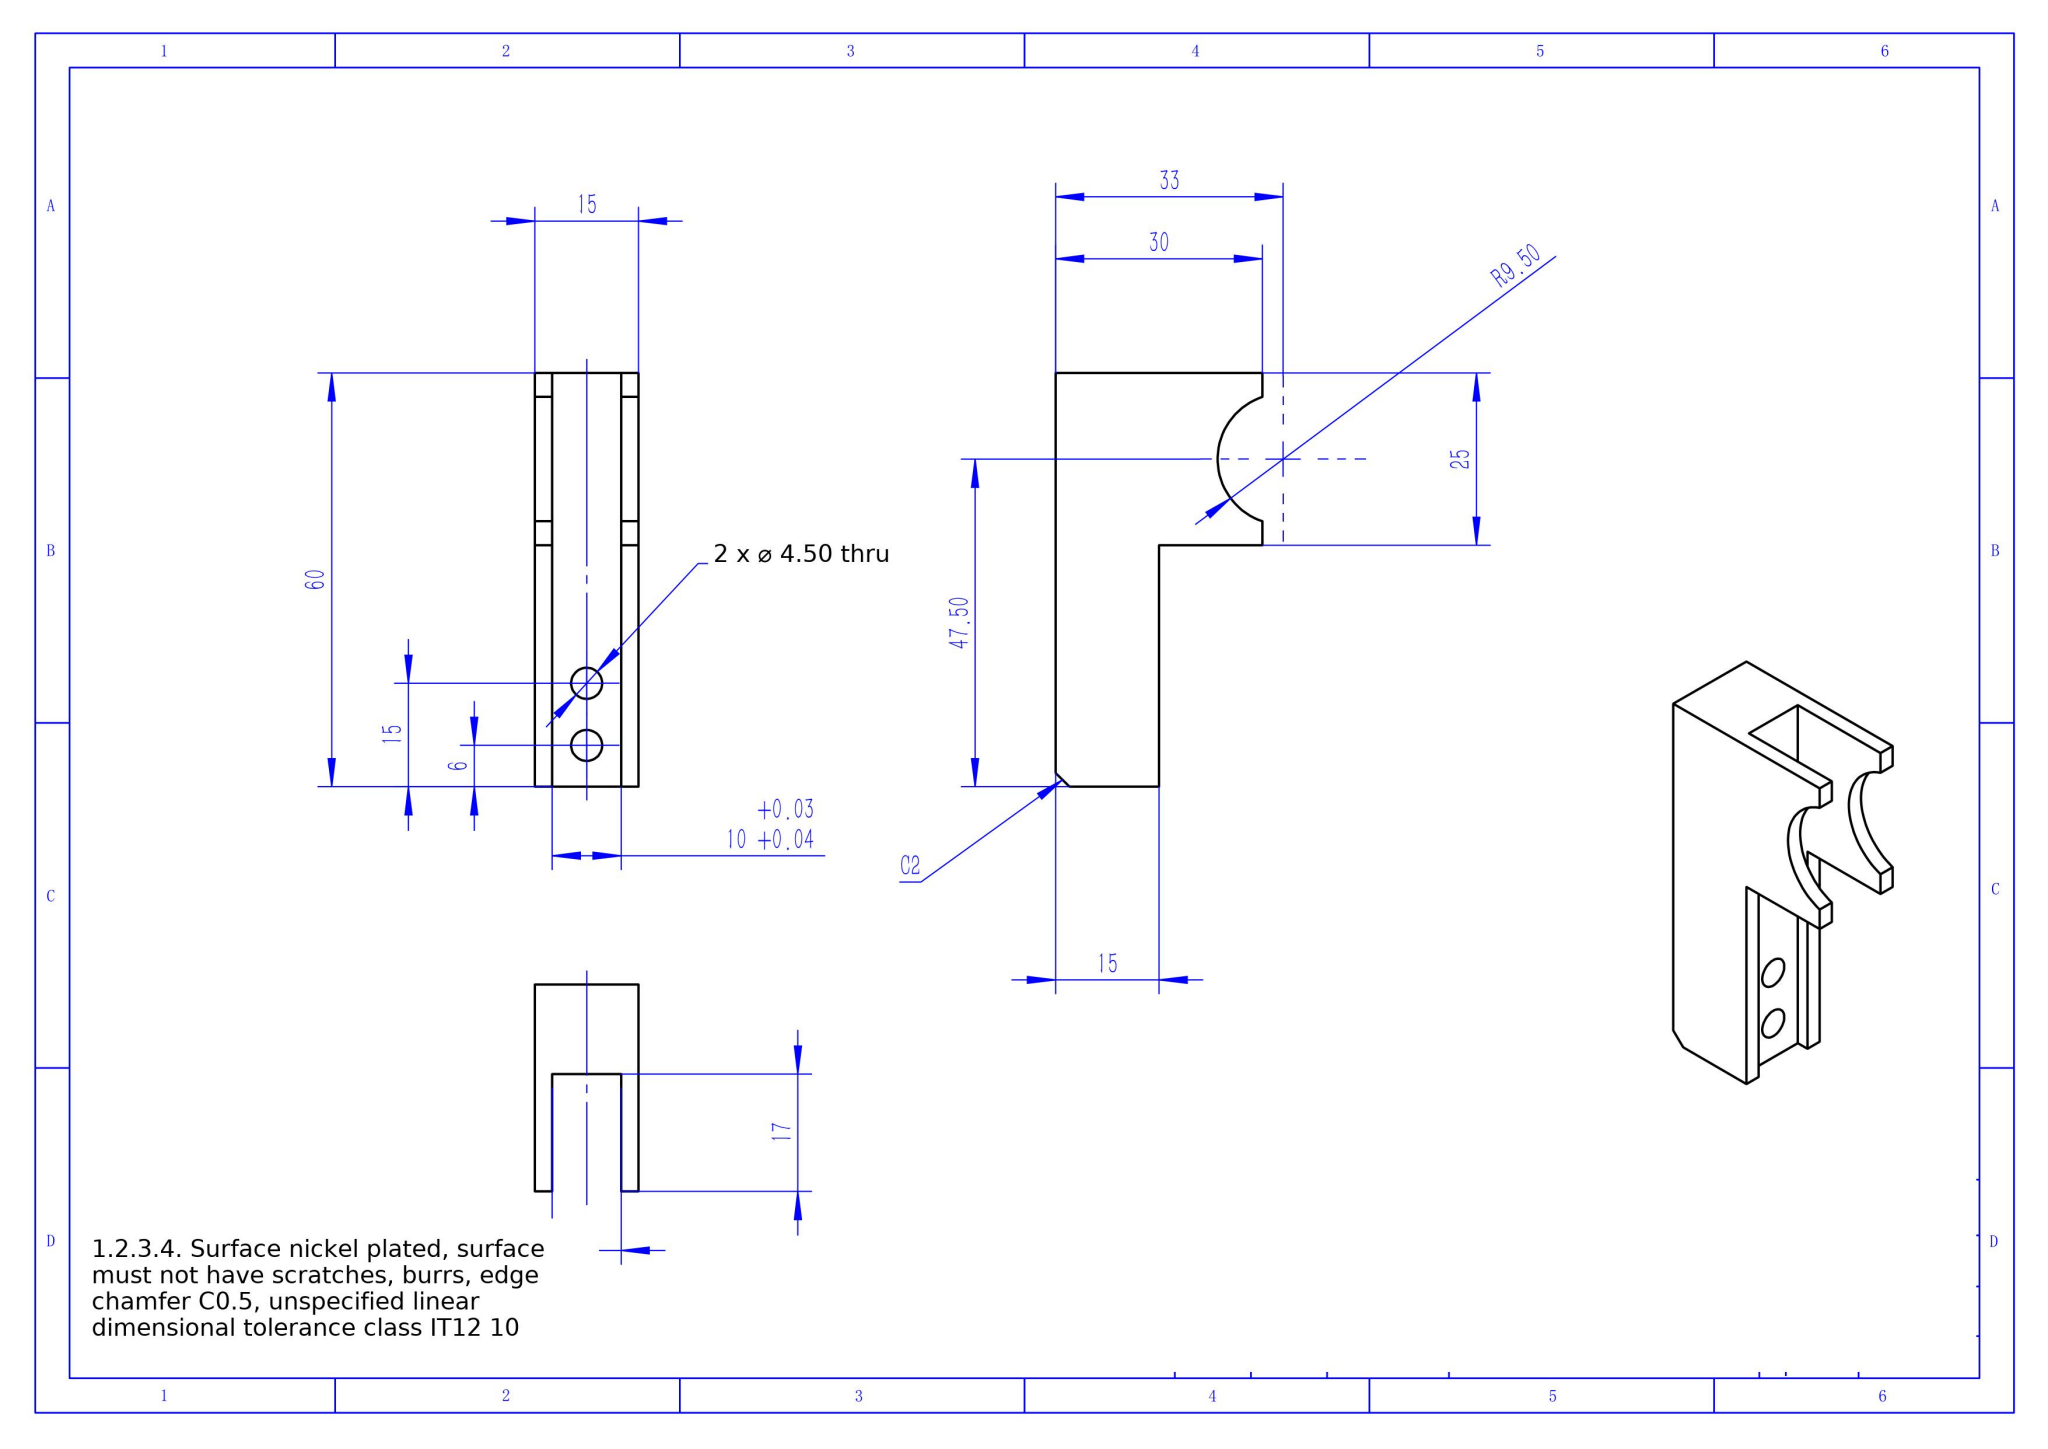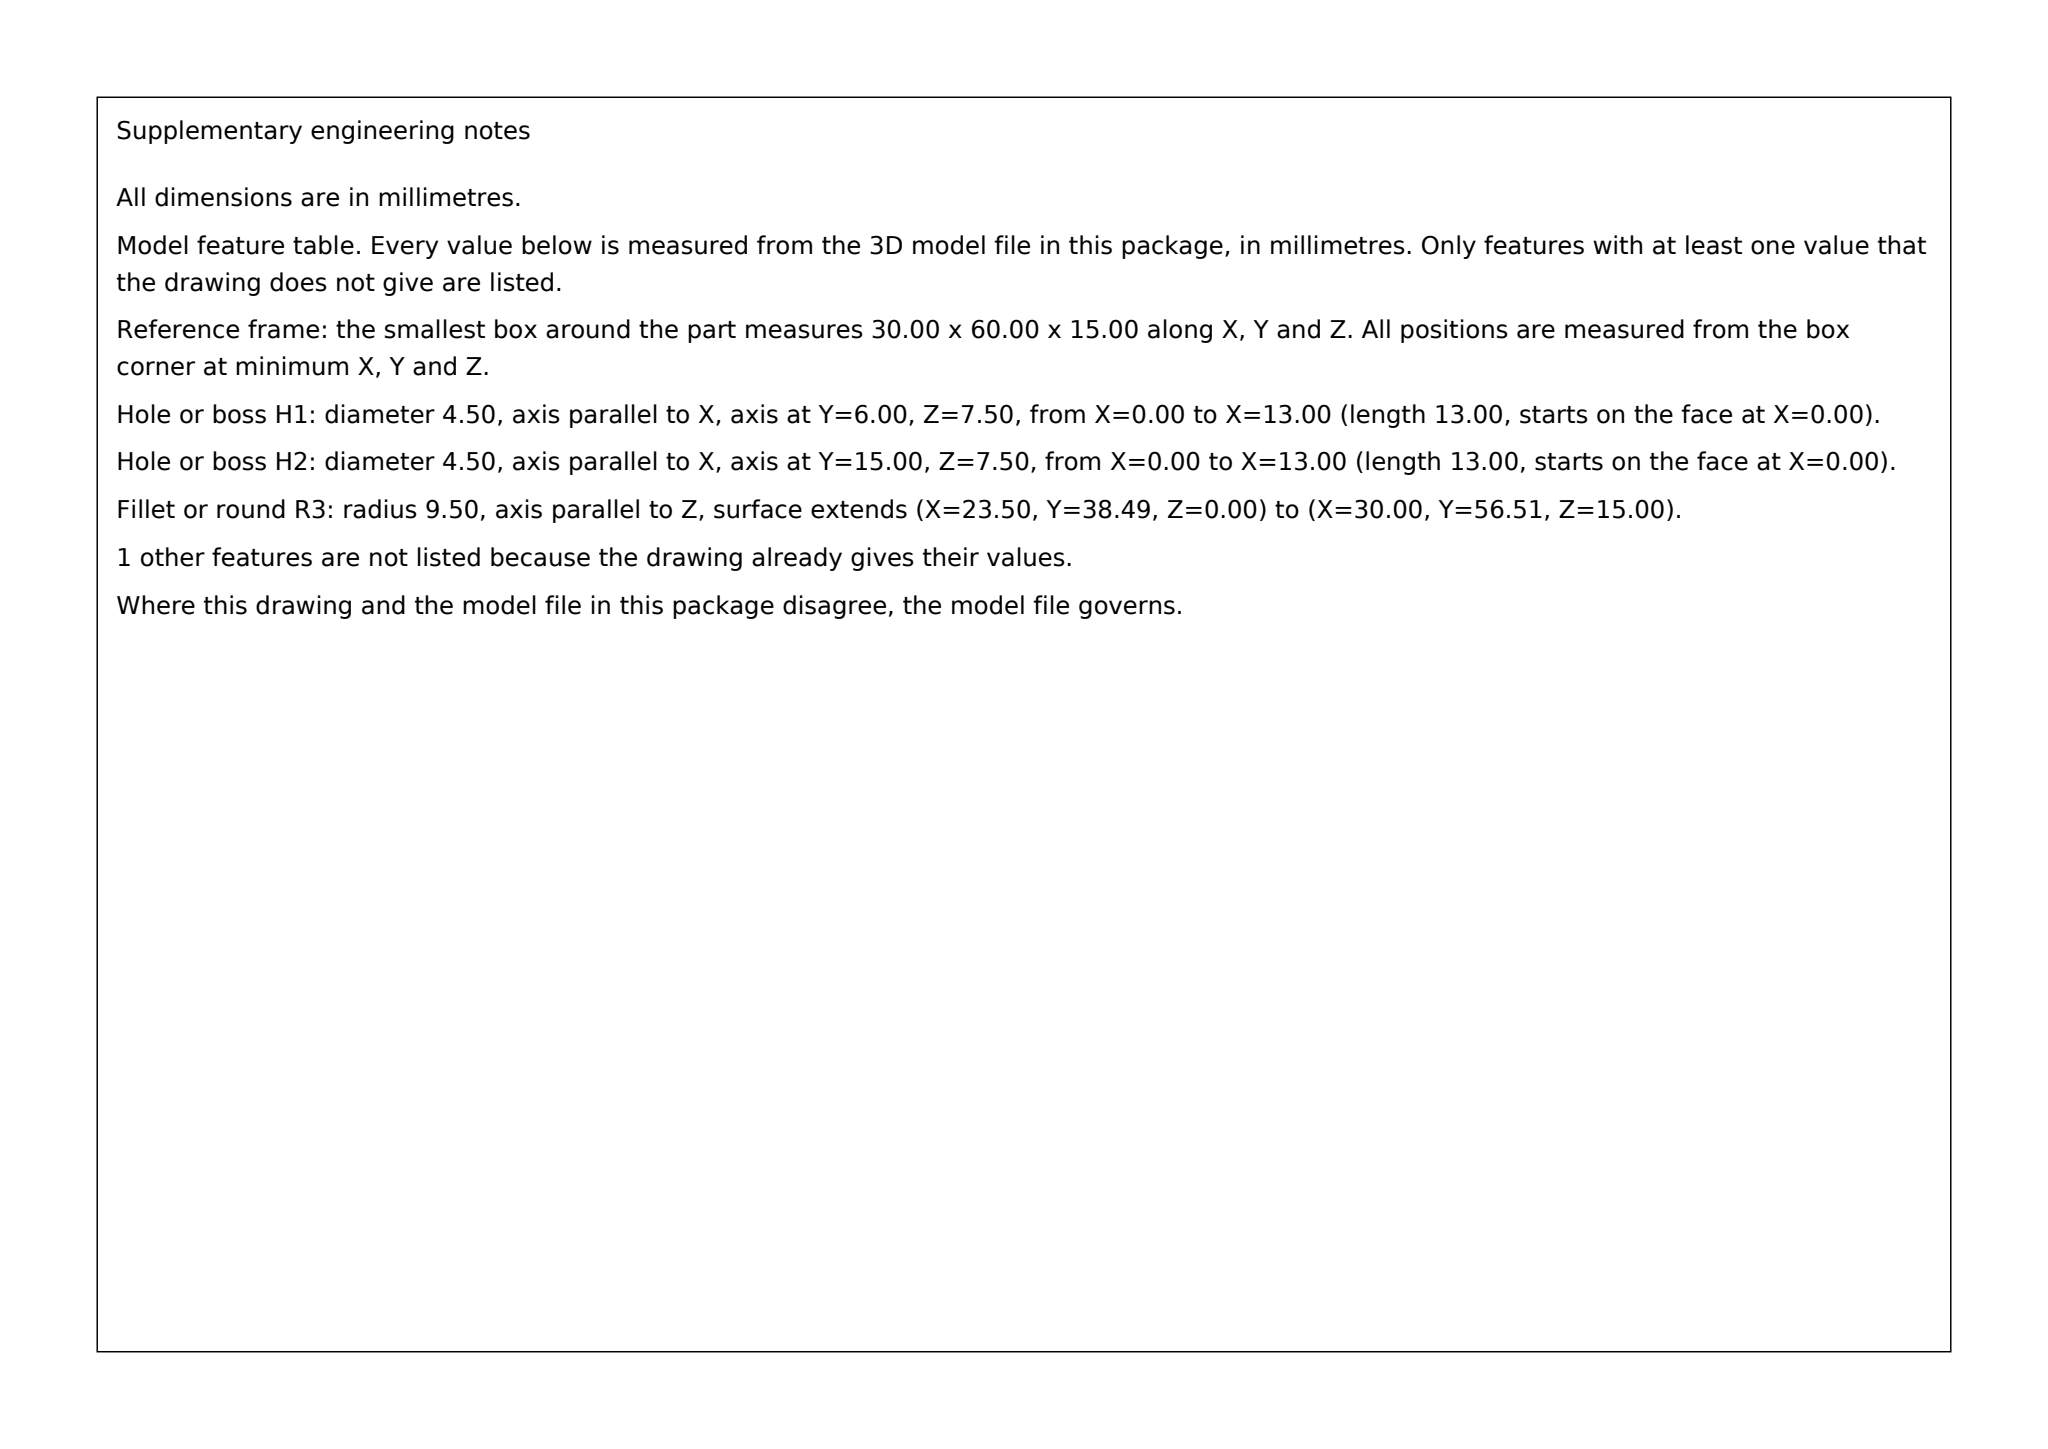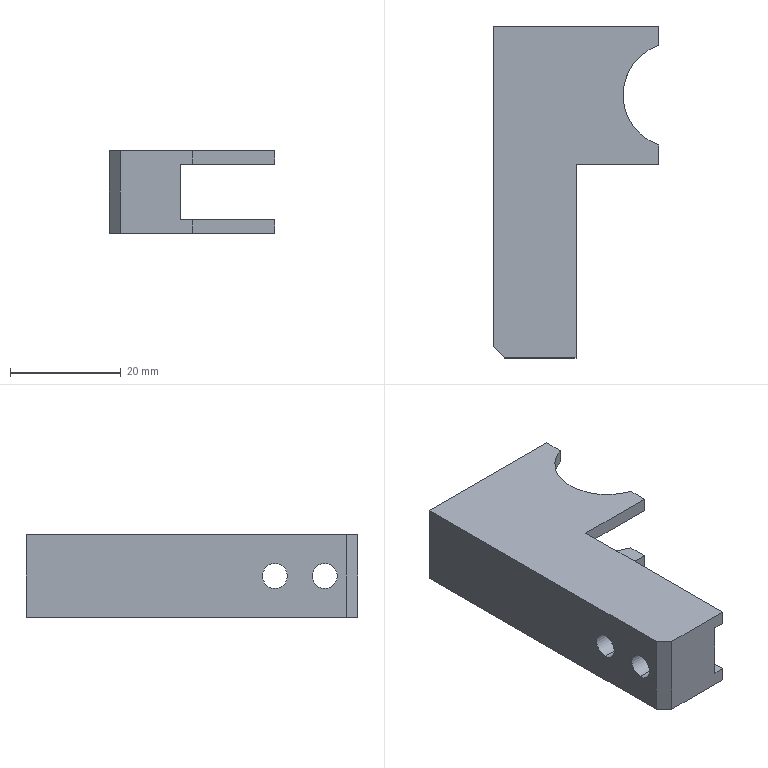Part | SolidWorks | mm | 1 solid | 25 faces | box 30 x 60 x 15 mm | volume 13303 mm3 | plane 17 | cylinder 8 | commonest cylinder face diameters 19 x4 4.5 x4
build123d program:
from build123d import *

# Parameters (mm, degrees)
BOSS_EXTRUDE1_DEPTH        = 15
F_4_5_4_5_DIAMETER_HOLE1_D = 4.5
CHAMFER1_SIZE              = 2
SKETCH5_W                  = 10
SKETCH5_H                  = 124.839
CUT_EXTRUDE2_DEPTH         = 17


with BuildPart() as part:
    # Sketch1 → Boss-Extrude1 (new body)
    with BuildSketch(Plane.XY):
        with BuildLine():
            Line((0, 0), (15, 0))
            Line((15, 0), (15, 35))
            Line((15, 35), (30, 35))
            Line((30, 35), (30, 38.486))
            ThreePointArc((30, 38.486), (23.5, 47.5), (30, 56.514))
            Line((30, 56.514), (30, 60))
            Line((30, 60), (0, 60))
            Line((0, 60), (0, 0))
        make_face()
    extrude(amount=BOSS_EXTRUDE1_DEPTH)

    # 4.5 _4.5_ Diameter Hole1 (through all)
    with Locations(Plane.ZY):
        with Locations((7.5, 6), (7.5, 15)):
            Hole(F_4_5_4_5_DIAMETER_HOLE1_D / 2)

    # Chamfer1
    chamfer1_edges = [part.edges().sort_by_distance(p)[0] for p in [
        (0, 0, 7.5),
    ]]
    chamfer(chamfer1_edges, length=CHAMFER1_SIZE)

    # Sketch5 → Cut-Extrude2 (cut)
    with BuildSketch(Plane(origin=(30, 0, 0), x_dir=(0, 0, -1), z_dir=(1, 0, 0))):
        with Locations((-7.5, 60)):
            Rectangle(SKETCH5_W, SKETCH5_H)
    extrude(amount=-CUT_EXTRUDE2_DEPTH, mode=Mode.SUBTRACT)


solid = part.part
STEP:
#1=CARTESIAN_POINT('',(23.5,47.5,15.));
#2=VERTEX_POINT('',#1);
#3=CARTESIAN_POINT('',(30.,56.514,15.));
#4=VERTEX_POINT('',#3);
#5=CARTESIAN_POINT('',(33.,47.5,15.));
#6=DIRECTION('',(0.,0.,-1.));
#7=DIRECTION('',(1.,0.,0.));
#8=AXIS2_PLACEMENT_3D('',#5,#6,#7);
#9=CIRCLE('',#8,9.5);
#10=EDGE_CURVE('',#2,#4,#9,.T.);
#11=ORIENTED_EDGE('',*,*,#10,.F.);
#12=CARTESIAN_POINT('',(23.5,47.5,12.5));
#13=VERTEX_POINT('',#12);
#14=CARTESIAN_POINT('',(23.5,47.5,15.));
#15=DIRECTION('',(0.,0.,-1.));
#16=VECTOR('',#15,1000.);
#17=LINE('',#14,#16);
#18=EDGE_CURVE('',#2,#13,#17,.T.);
#19=ORIENTED_EDGE('',*,*,#18,.T.);
#20=CARTESIAN_POINT('',(30.,56.514,12.5));
#21=VERTEX_POINT('',#20);
#22=CARTESIAN_POINT('',(33.,47.5,12.5));
#23=DIRECTION('',(0.,0.,-1.));
#24=DIRECTION('',(1.,-0.,0.));
#25=AXIS2_PLACEMENT_3D('',#22,#23,#24);
#26=CIRCLE('',#25,9.5);
#27=EDGE_CURVE('',#13,#21,#26,.T.);
#28=ORIENTED_EDGE('',*,*,#27,.T.);
#29=CARTESIAN_POINT('',(30.,56.514,15.));
#30=DIRECTION('',(0.,0.,-1.));
#31=VECTOR('',#30,1000.);
#32=LINE('',#29,#31);
#33=EDGE_CURVE('',#4,#21,#32,.T.);
#34=ORIENTED_EDGE('',*,*,#33,.F.);
#35=EDGE_LOOP('',(#11,#19,#28,#34));
#36=FACE_OUTER_BOUND('',#35,.T.);
#37=CARTESIAN_POINT('',(33.,47.5,15.));
#38=DIRECTION('',(0.,0.,-1.));
#39=DIRECTION('',(-1.,0.,0.));
#40=AXIS2_PLACEMENT_3D('',#37,#38,#39);
#41=CYLINDRICAL_SURFACE('',#40,9.5);
#42=ADVANCED_FACE('',(#36),#41,.F.);
#43=CARTESIAN_POINT('',(13.,6.,5.25));
#44=VERTEX_POINT('',#43);
#45=CARTESIAN_POINT('',(13.,6.,9.75));
#46=VERTEX_POINT('',#45);
#47=CARTESIAN_POINT('',(13.,6.,7.5));
#48=DIRECTION('',(-1.,0.,0.));
#49=DIRECTION('',(0.,0.,-1.));
#50=AXIS2_PLACEMENT_3D('',#47,#48,#49);
#51=CIRCLE('',#50,2.25);
#52=EDGE_CURVE('',#44,#46,#51,.T.);
#53=ORIENTED_EDGE('',*,*,#52,.F.);
#54=CARTESIAN_POINT('',(-0.,6.,5.25));
#55=VERTEX_POINT('',#54);
#56=CARTESIAN_POINT('',(0.,6.,5.25));
#57=DIRECTION('',(-1.,0.,0.));
#58=VECTOR('',#57,1000.);
#59=LINE('',#56,#58);
#60=EDGE_CURVE('',#44,#55,#59,.T.);
#61=ORIENTED_EDGE('',*,*,#60,.T.);
#62=CARTESIAN_POINT('',(-0.,6.,9.75));
#63=VERTEX_POINT('',#62);
#64=CARTESIAN_POINT('',(-0.,6.,7.5));
#65=DIRECTION('',(-1.,0.,0.));
#66=DIRECTION('',(0.,0.,1.));
#67=AXIS2_PLACEMENT_3D('',#64,#65,#66);
#68=CIRCLE('',#67,2.25);
#69=EDGE_CURVE('',#55,#63,#68,.T.);
#70=ORIENTED_EDGE('',*,*,#69,.T.);
#71=CARTESIAN_POINT('',(0.,6.,9.75));
#72=DIRECTION('',(-1.,0.,0.));
#73=VECTOR('',#72,1000.);
#74=LINE('',#71,#73);
#75=EDGE_CURVE('',#46,#63,#74,.T.);
#76=ORIENTED_EDGE('',*,*,#75,.F.);
#77=EDGE_LOOP('',(#53,#61,#70,#76));
#78=FACE_OUTER_BOUND('',#77,.T.);
#79=CARTESIAN_POINT('',(0.,6.,7.5));
#80=DIRECTION('',(-1.,0.,0.));
#81=DIRECTION('',(0.,0.,1.));
#82=AXIS2_PLACEMENT_3D('',#79,#80,#81);
#83=CYLINDRICAL_SURFACE('',#82,2.25);
#84=ADVANCED_FACE('',(#78),#83,.F.);
#85=CARTESIAN_POINT('',(13.,15.,5.25));
#86=VERTEX_POINT('',#85);
#87=CARTESIAN_POINT('',(13.,15.,9.75));
#88=VERTEX_POINT('',#87);
#89=CARTESIAN_POINT('',(13.,15.,7.5));
#90=DIRECTION('',(-1.,0.,0.));
#91=DIRECTION('',(0.,0.,-1.));
#92=AXIS2_PLACEMENT_3D('',#89,#90,#91);
#93=CIRCLE('',#92,2.25);
#94=EDGE_CURVE('',#86,#88,#93,.T.);
#95=ORIENTED_EDGE('',*,*,#94,.F.);
#96=CARTESIAN_POINT('',(-0.,15.,5.25));
#97=VERTEX_POINT('',#96);
#98=CARTESIAN_POINT('',(0.,15.,5.25));
#99=DIRECTION('',(-1.,0.,0.));
#100=VECTOR('',#99,1000.);
#101=LINE('',#98,#100);
#102=EDGE_CURVE('',#86,#97,#101,.T.);
#103=ORIENTED_EDGE('',*,*,#102,.T.);
#104=CARTESIAN_POINT('',(-0.,15.,9.75));
#105=VERTEX_POINT('',#104);
#106=CARTESIAN_POINT('',(-0.,15.,7.5));
#107=DIRECTION('',(-1.,0.,0.));
#108=DIRECTION('',(0.,0.,1.));
#109=AXIS2_PLACEMENT_3D('',#106,#107,#108);
#110=CIRCLE('',#109,2.25);
#111=EDGE_CURVE('',#97,#105,#110,.T.);
#112=ORIENTED_EDGE('',*,*,#111,.T.);
#113=CARTESIAN_POINT('',(0.,15.,9.75));
#114=DIRECTION('',(-1.,0.,0.));
#115=VECTOR('',#114,1000.);
#116=LINE('',#113,#115);
#117=EDGE_CURVE('',#88,#105,#116,.T.);
#118=ORIENTED_EDGE('',*,*,#117,.F.);
#119=EDGE_LOOP('',(#95,#103,#112,#118));
#120=FACE_OUTER_BOUND('',#119,.T.);
#121=CARTESIAN_POINT('',(0.,15.,7.5));
#122=DIRECTION('',(-1.,0.,0.));
#123=DIRECTION('',(0.,0.,1.));
#124=AXIS2_PLACEMENT_3D('',#121,#122,#123);
#125=CYLINDRICAL_SURFACE('',#124,2.25);
#126=ADVANCED_FACE('',(#120),#125,.F.);
#127=CARTESIAN_POINT('',(30.,56.514,2.5));
#128=VERTEX_POINT('',#127);
#129=CARTESIAN_POINT('',(23.5,47.5,2.5));
#130=VERTEX_POINT('',#129);
#131=CARTESIAN_POINT('',(33.,47.5,2.5));
#132=DIRECTION('',(0.,0.,1.));
#133=DIRECTION('',(-1.,0.,0.));
#134=AXIS2_PLACEMENT_3D('',#131,#132,#133);
#135=CIRCLE('',#134,9.5);
#136=EDGE_CURVE('',#128,#130,#135,.T.);
#137=ORIENTED_EDGE('',*,*,#136,.T.);
#138=CARTESIAN_POINT('',(23.5,47.5,0.));
#139=VERTEX_POINT('',#138);
#140=CARTESIAN_POINT('',(23.5,47.5,15.));
#141=DIRECTION('',(0.,0.,-1.));
#142=VECTOR('',#141,1000.);
#143=LINE('',#140,#142);
#144=EDGE_CURVE('',#130,#139,#143,.T.);
#145=ORIENTED_EDGE('',*,*,#144,.T.);
#146=CARTESIAN_POINT('',(30.,56.514,0.));
#147=VERTEX_POINT('',#146);
#148=CARTESIAN_POINT('',(33.,47.5,0.));
#149=DIRECTION('',(0.,0.,-1.));
#150=DIRECTION('',(1.,0.,0.));
#151=AXIS2_PLACEMENT_3D('',#148,#149,#150);
#152=CIRCLE('',#151,9.5);
#153=EDGE_CURVE('',#139,#147,#152,.T.);
#154=ORIENTED_EDGE('',*,*,#153,.T.);
#155=CARTESIAN_POINT('',(30.,56.514,15.));
#156=DIRECTION('',(0.,0.,-1.));
#157=VECTOR('',#156,1000.);
#158=LINE('',#155,#157);
#159=EDGE_CURVE('',#128,#147,#158,.T.);
#160=ORIENTED_EDGE('',*,*,#159,.F.);
#161=EDGE_LOOP('',(#137,#145,#154,#160));
#162=FACE_OUTER_BOUND('',#161,.T.);
#163=CARTESIAN_POINT('',(33.,47.5,15.));
#164=DIRECTION('',(0.,0.,-1.));
#165=DIRECTION('',(-1.,0.,0.));
#166=AXIS2_PLACEMENT_3D('',#163,#164,#165);
#167=CYLINDRICAL_SURFACE('',#166,9.5);
#168=ADVANCED_FACE('',(#162),#167,.F.);
#169=CARTESIAN_POINT('',(15.,35.,2.5));
#170=VERTEX_POINT('',#169);
#171=CARTESIAN_POINT('',(15.,35.,0.));
#172=VERTEX_POINT('',#171);
#173=CARTESIAN_POINT('',(15.,35.,15.));
#174=DIRECTION('',(0.,0.,-1.));
#175=VECTOR('',#174,1000.);
#176=LINE('',#173,#175);
#177=EDGE_CURVE('',#170,#172,#176,.T.);
#178=ORIENTED_EDGE('',*,*,#177,.F.);
#179=CARTESIAN_POINT('',(15.,0.,2.5));
#180=VERTEX_POINT('',#179);
#181=CARTESIAN_POINT('',(15.,35.,2.5));
#182=DIRECTION('',(0.,-1.,0.));
#183=VECTOR('',#182,1000.);
#184=LINE('',#181,#183);
#185=EDGE_CURVE('',#170,#180,#184,.T.);
#186=ORIENTED_EDGE('',*,*,#185,.T.);
#187=CARTESIAN_POINT('',(15.,0.,0.));
#188=VERTEX_POINT('',#187);
#189=CARTESIAN_POINT('',(15.,0.,15.));
#190=DIRECTION('',(0.,0.,-1.));
#191=VECTOR('',#190,1000.);
#192=LINE('',#189,#191);
#193=EDGE_CURVE('',#180,#188,#192,.T.);
#194=ORIENTED_EDGE('',*,*,#193,.T.);
#195=CARTESIAN_POINT('',(15.,35.,0.));
#196=DIRECTION('',(-0.,1.,0.));
#197=VECTOR('',#196,1000.);
#198=LINE('',#195,#197);
#199=EDGE_CURVE('',#188,#172,#198,.T.);
#200=ORIENTED_EDGE('',*,*,#199,.T.);
#201=EDGE_LOOP('',(#178,#186,#194,#200));
#202=FACE_OUTER_BOUND('',#201,.T.);
#203=CARTESIAN_POINT('',(15.,35.,15.));
#204=DIRECTION('',(-1.,-0.,0.));
#205=DIRECTION('',(0.,-1.,0.));
#206=AXIS2_PLACEMENT_3D('',#203,#204,#205);
#207=PLANE('',#206);
#208=ADVANCED_FACE('',(#202),#207,.F.);
#209=CARTESIAN_POINT('',(30.,35.,2.5));
#210=VERTEX_POINT('',#209);
#211=CARTESIAN_POINT('',(30.,35.,0.));
#212=VERTEX_POINT('',#211);
#213=CARTESIAN_POINT('',(30.,35.,15.));
#214=DIRECTION('',(0.,0.,-1.));
#215=VECTOR('',#214,1000.);
#216=LINE('',#213,#215);
#217=EDGE_CURVE('',#210,#212,#216,.T.);
#218=ORIENTED_EDGE('',*,*,#217,.F.);
#219=CARTESIAN_POINT('',(30.,35.,2.5));
#220=DIRECTION('',(-1.,0.,0.));
#221=VECTOR('',#220,1000.);
#222=LINE('',#219,#221);
#223=EDGE_CURVE('',#210,#170,#222,.T.);
#224=ORIENTED_EDGE('',*,*,#223,.T.);
#225=ORIENTED_EDGE('',*,*,#177,.T.);
#226=CARTESIAN_POINT('',(30.,35.,0.));
#227=DIRECTION('',(1.,0.,0.));
#228=VECTOR('',#227,1000.);
#229=LINE('',#226,#228);
#230=EDGE_CURVE('',#172,#212,#229,.T.);
#231=ORIENTED_EDGE('',*,*,#230,.T.);
#232=EDGE_LOOP('',(#218,#224,#225,#231));
#233=FACE_OUTER_BOUND('',#232,.T.);
#234=CARTESIAN_POINT('',(30.,35.,15.));
#235=DIRECTION('',(0.,1.,0.));
#236=DIRECTION('',(0.,0.,1.));
#237=AXIS2_PLACEMENT_3D('',#234,#235,#236);
#238=PLANE('',#237);
#239=ADVANCED_FACE('',(#233),#238,.F.);
#240=CARTESIAN_POINT('',(30.,38.486,2.5));
#241=VERTEX_POINT('',#240);
#242=CARTESIAN_POINT('',(30.,38.486,0.));
#243=VERTEX_POINT('',#242);
#244=CARTESIAN_POINT('',(30.,38.486,15.));
#245=DIRECTION('',(0.,0.,-1.));
#246=VECTOR('',#245,1000.);
#247=LINE('',#244,#246);
#248=EDGE_CURVE('',#241,#243,#247,.T.);
#249=ORIENTED_EDGE('',*,*,#248,.F.);
#250=CARTESIAN_POINT('',(30.,122.42,2.5));
#251=DIRECTION('',(0.,1.,0.));
#252=VECTOR('',#251,1000.);
#253=LINE('',#250,#252);
#254=EDGE_CURVE('',#210,#241,#253,.T.);
#255=ORIENTED_EDGE('',*,*,#254,.F.);
#256=ORIENTED_EDGE('',*,*,#217,.T.);
#257=CARTESIAN_POINT('',(30.,38.486,0.));
#258=DIRECTION('',(0.,1.,0.));
#259=VECTOR('',#258,1000.);
#260=LINE('',#257,#259);
#261=EDGE_CURVE('',#212,#243,#260,.T.);
#262=ORIENTED_EDGE('',*,*,#261,.T.);
#263=EDGE_LOOP('',(#249,#255,#256,#262));
#264=FACE_OUTER_BOUND('',#263,.T.);
#265=CARTESIAN_POINT('',(30.,38.486,15.));
#266=DIRECTION('',(-1.,0.,0.));
#267=DIRECTION('',(0.,0.,1.));
#268=AXIS2_PLACEMENT_3D('',#265,#266,#267);
#269=PLANE('',#268);
#270=ADVANCED_FACE('',(#264),#269,.F.);
#271=ORIENTED_EDGE('',*,*,#144,.F.);
#272=CARTESIAN_POINT('',(33.,47.5,2.5));
#273=DIRECTION('',(0.,0.,1.));
#274=DIRECTION('',(-1.,0.,0.));
#275=AXIS2_PLACEMENT_3D('',#272,#273,#274);
#276=CIRCLE('',#275,9.5);
#277=EDGE_CURVE('',#130,#241,#276,.T.);
#278=ORIENTED_EDGE('',*,*,#277,.T.);
#279=ORIENTED_EDGE('',*,*,#248,.T.);
#280=CARTESIAN_POINT('',(33.,47.5,0.));
#281=DIRECTION('',(0.,0.,-1.));
#282=DIRECTION('',(1.,0.,0.));
#283=AXIS2_PLACEMENT_3D('',#280,#281,#282);
#284=CIRCLE('',#283,9.5);
#285=EDGE_CURVE('',#243,#139,#284,.T.);
#286=ORIENTED_EDGE('',*,*,#285,.T.);
#287=EDGE_LOOP('',(#271,#278,#279,#286));
#288=FACE_OUTER_BOUND('',#287,.T.);
#289=CARTESIAN_POINT('',(33.,47.5,15.));
#290=DIRECTION('',(0.,0.,-1.));
#291=DIRECTION('',(-1.,0.,0.));
#292=AXIS2_PLACEMENT_3D('',#289,#290,#291);
#293=CYLINDRICAL_SURFACE('',#292,9.5);
#294=ADVANCED_FACE('',(#288),#293,.F.);
#295=CARTESIAN_POINT('',(30.,60.,2.5));
#296=VERTEX_POINT('',#295);
#297=CARTESIAN_POINT('',(30.,60.,0.));
#298=VERTEX_POINT('',#297);
#299=CARTESIAN_POINT('',(30.,60.,15.));
#300=DIRECTION('',(0.,0.,-1.));
#301=VECTOR('',#300,1000.);
#302=LINE('',#299,#301);
#303=EDGE_CURVE('',#296,#298,#302,.T.);
#304=ORIENTED_EDGE('',*,*,#303,.F.);
#305=CARTESIAN_POINT('',(30.,122.42,2.5));
#306=DIRECTION('',(0.,1.,0.));
#307=VECTOR('',#306,1000.);
#308=LINE('',#305,#307);
#309=EDGE_CURVE('',#128,#296,#308,.T.);
#310=ORIENTED_EDGE('',*,*,#309,.F.);
#311=ORIENTED_EDGE('',*,*,#159,.T.);
#312=CARTESIAN_POINT('',(30.,60.,0.));
#313=DIRECTION('',(0.,1.,0.));
#314=VECTOR('',#313,1000.);
#315=LINE('',#312,#314);
#316=EDGE_CURVE('',#147,#298,#315,.T.);
#317=ORIENTED_EDGE('',*,*,#316,.T.);
#318=EDGE_LOOP('',(#304,#310,#311,#317));
#319=FACE_OUTER_BOUND('',#318,.T.);
#320=CARTESIAN_POINT('',(30.,60.,15.));
#321=DIRECTION('',(-1.,0.,0.));
#322=DIRECTION('',(0.,0.,1.));
#323=AXIS2_PLACEMENT_3D('',#320,#321,#322);
#324=PLANE('',#323);
#325=ADVANCED_FACE('',(#319),#324,.F.);
#326=ORIENTED_EDGE('',*,*,#102,.F.);
#327=CARTESIAN_POINT('',(13.,15.,7.5));
#328=DIRECTION('',(-1.,0.,0.));
#329=DIRECTION('',(0.,0.,-1.));
#330=AXIS2_PLACEMENT_3D('',#327,#328,#329);
#331=CIRCLE('',#330,2.25);
#332=EDGE_CURVE('',#88,#86,#331,.T.);
#333=ORIENTED_EDGE('',*,*,#332,.F.);
#334=ORIENTED_EDGE('',*,*,#117,.T.);
#335=CARTESIAN_POINT('',(-0.,15.,7.5));
#336=DIRECTION('',(-1.,0.,0.));
#337=DIRECTION('',(0.,0.,1.));
#338=AXIS2_PLACEMENT_3D('',#335,#336,#337);
#339=CIRCLE('',#338,2.25);
#340=EDGE_CURVE('',#105,#97,#339,.T.);
#341=ORIENTED_EDGE('',*,*,#340,.T.);
#342=EDGE_LOOP('',(#326,#333,#334,#341));
#343=FACE_OUTER_BOUND('',#342,.T.);
#344=CARTESIAN_POINT('',(0.,15.,7.5));
#345=DIRECTION('',(-1.,0.,0.));
#346=DIRECTION('',(0.,0.,1.));
#347=AXIS2_PLACEMENT_3D('',#344,#345,#346);
#348=CYLINDRICAL_SURFACE('',#347,2.25);
#349=ADVANCED_FACE('',(#343),#348,.F.);
#350=ORIENTED_EDGE('',*,*,#60,.F.);
#351=CARTESIAN_POINT('',(13.,6.,7.5));
#352=DIRECTION('',(-1.,0.,0.));
#353=DIRECTION('',(0.,0.,-1.));
#354=AXIS2_PLACEMENT_3D('',#351,#352,#353);
#355=CIRCLE('',#354,2.25);
#356=EDGE_CURVE('',#46,#44,#355,.T.);
#357=ORIENTED_EDGE('',*,*,#356,.F.);
#358=ORIENTED_EDGE('',*,*,#75,.T.);
#359=CARTESIAN_POINT('',(-0.,6.,7.5));
#360=DIRECTION('',(-1.,0.,0.));
#361=DIRECTION('',(0.,0.,1.));
#362=AXIS2_PLACEMENT_3D('',#359,#360,#361);
#363=CIRCLE('',#362,2.25);
#364=EDGE_CURVE('',#63,#55,#363,.T.);
#365=ORIENTED_EDGE('',*,*,#364,.T.);
#366=EDGE_LOOP('',(#350,#357,#358,#365));
#367=FACE_OUTER_BOUND('',#366,.T.);
#368=CARTESIAN_POINT('',(0.,6.,7.5));
#369=DIRECTION('',(-1.,0.,0.));
#370=DIRECTION('',(0.,0.,1.));
#371=AXIS2_PLACEMENT_3D('',#368,#369,#370);
#372=CYLINDRICAL_SURFACE('',#371,2.25);
#373=ADVANCED_FACE('',(#367),#372,.F.);
#374=CARTESIAN_POINT('',(0.,60.,0.));
#375=VERTEX_POINT('',#374);
#376=CARTESIAN_POINT('',(0.,2.,0.));
#377=VERTEX_POINT('',#376);
#378=CARTESIAN_POINT('',(0.,0.,0.));
#379=DIRECTION('',(0.,-1.,0.));
#380=VECTOR('',#379,1000.);
#381=LINE('',#378,#380);
#382=EDGE_CURVE('',#375,#377,#381,.T.);
#383=ORIENTED_EDGE('',*,*,#382,.T.);
#384=CARTESIAN_POINT('',(0.,2.,15.));
#385=VERTEX_POINT('',#384);
#386=CARTESIAN_POINT('',(0.,2.,15.));
#387=DIRECTION('',(0.,0.,1.));
#388=VECTOR('',#387,1000.);
#389=LINE('',#386,#388);
#390=EDGE_CURVE('',#377,#385,#389,.T.);
#391=ORIENTED_EDGE('',*,*,#390,.T.);
#392=CARTESIAN_POINT('',(0.,60.,15.));
#393=VERTEX_POINT('',#392);
#394=CARTESIAN_POINT('',(0.,0.,15.));
#395=DIRECTION('',(0.,-1.,0.));
#396=VECTOR('',#395,1000.);
#397=LINE('',#394,#396);
#398=EDGE_CURVE('',#393,#385,#397,.T.);
#399=ORIENTED_EDGE('',*,*,#398,.F.);
#400=CARTESIAN_POINT('',(0.,60.,15.));
#401=DIRECTION('',(0.,0.,-1.));
#402=VECTOR('',#401,1000.);
#403=LINE('',#400,#402);
#404=EDGE_CURVE('',#393,#375,#403,.T.);
#405=ORIENTED_EDGE('',*,*,#404,.T.);
#406=EDGE_LOOP('',(#383,#391,#399,#405));
#407=FACE_OUTER_BOUND('',#406,.T.);
#408=ORIENTED_EDGE('',*,*,#340,.F.);
#409=ORIENTED_EDGE('',*,*,#111,.F.);
#410=EDGE_LOOP('',(#408,#409));
#411=FACE_BOUND('',#410,.T.);
#412=ORIENTED_EDGE('',*,*,#364,.F.);
#413=ORIENTED_EDGE('',*,*,#69,.F.);
#414=EDGE_LOOP('',(#412,#413));
#415=FACE_BOUND('',#414,.T.);
#416=CARTESIAN_POINT('',(0.,0.,15.));
#417=DIRECTION('',(1.,0.,0.));
#418=DIRECTION('',(0.,0.,-1.));
#419=AXIS2_PLACEMENT_3D('',#416,#417,#418);
#420=PLANE('',#419);
#421=ADVANCED_FACE('',(#407,#411,#415),#420,.F.);
#422=ORIENTED_EDGE('',*,*,#193,.F.);
#423=CARTESIAN_POINT('',(13.,0.,2.5));
#424=VERTEX_POINT('',#423);
#425=CARTESIAN_POINT('',(0.,0.,2.5));
#426=DIRECTION('',(-1.,0.,0.));
#427=VECTOR('',#426,1000.);
#428=LINE('',#425,#427);
#429=EDGE_CURVE('',#180,#424,#428,.T.);
#430=ORIENTED_EDGE('',*,*,#429,.T.);
#431=CARTESIAN_POINT('',(13.,0.,12.5));
#432=VERTEX_POINT('',#431);
#433=CARTESIAN_POINT('',(13.,0.,15.));
#434=DIRECTION('',(0.,0.,-1.));
#435=VECTOR('',#434,1000.);
#436=LINE('',#433,#435);
#437=EDGE_CURVE('',#432,#424,#436,.T.);
#438=ORIENTED_EDGE('',*,*,#437,.F.);
#439=CARTESIAN_POINT('',(15.,0.,12.5));
#440=VERTEX_POINT('',#439);
#441=CARTESIAN_POINT('',(0.,0.,12.5));
#442=DIRECTION('',(1.,0.,0.));
#443=VECTOR('',#442,1000.);
#444=LINE('',#441,#443);
#445=EDGE_CURVE('',#432,#440,#444,.T.);
#446=ORIENTED_EDGE('',*,*,#445,.T.);
#447=CARTESIAN_POINT('',(15.,0.,15.));
#448=VERTEX_POINT('',#447);
#449=CARTESIAN_POINT('',(15.,0.,15.));
#450=DIRECTION('',(0.,0.,-1.));
#451=VECTOR('',#450,1000.);
#452=LINE('',#449,#451);
#453=EDGE_CURVE('',#448,#440,#452,.T.);
#454=ORIENTED_EDGE('',*,*,#453,.F.);
#455=CARTESIAN_POINT('',(2.,0.,15.));
#456=VERTEX_POINT('',#455);
#457=CARTESIAN_POINT('',(0.,0.,15.));
#458=DIRECTION('',(1.,0.,0.));
#459=VECTOR('',#458,1000.);
#460=LINE('',#457,#459);
#461=EDGE_CURVE('',#456,#448,#460,.T.);
#462=ORIENTED_EDGE('',*,*,#461,.F.);
#463=CARTESIAN_POINT('',(2.,0.,0.));
#464=VERTEX_POINT('',#463);
#465=CARTESIAN_POINT('',(2.,0.,15.));
#466=DIRECTION('',(0.,0.,-1.));
#467=VECTOR('',#466,1000.);
#468=LINE('',#465,#467);
#469=EDGE_CURVE('',#456,#464,#468,.T.);
#470=ORIENTED_EDGE('',*,*,#469,.T.);
#471=CARTESIAN_POINT('',(0.,0.,0.));
#472=DIRECTION('',(1.,0.,0.));
#473=VECTOR('',#472,1000.);
#474=LINE('',#471,#473);
#475=EDGE_CURVE('',#464,#188,#474,.T.);
#476=ORIENTED_EDGE('',*,*,#475,.T.);
#477=EDGE_LOOP('',(#422,#430,#438,#446,#454,#462,#470,#476));
#478=FACE_OUTER_BOUND('',#477,.T.);
#479=CARTESIAN_POINT('',(0.,0.,15.));
#480=DIRECTION('',(0.,1.,0.));
#481=DIRECTION('',(0.,0.,1.));
#482=AXIS2_PLACEMENT_3D('',#479,#480,#481);
#483=PLANE('',#482);
#484=ADVANCED_FACE('',(#478),#483,.F.);
#485=ORIENTED_EDGE('',*,*,#453,.T.);
#486=CARTESIAN_POINT('',(15.,35.,12.5));
#487=VERTEX_POINT('',#486);
#488=CARTESIAN_POINT('',(15.,35.,12.5));
#489=DIRECTION('',(-0.,1.,0.));
#490=VECTOR('',#489,1000.);
#491=LINE('',#488,#490);
#492=EDGE_CURVE('',#440,#487,#491,.T.);
#493=ORIENTED_EDGE('',*,*,#492,.T.);
#494=CARTESIAN_POINT('',(15.,35.,15.));
#495=VERTEX_POINT('',#494);
#496=CARTESIAN_POINT('',(15.,35.,15.));
#497=DIRECTION('',(0.,0.,-1.));
#498=VECTOR('',#497,1000.);
#499=LINE('',#496,#498);
#500=EDGE_CURVE('',#495,#487,#499,.T.);
#501=ORIENTED_EDGE('',*,*,#500,.F.);
#502=CARTESIAN_POINT('',(15.,35.,15.));
#503=DIRECTION('',(-0.,1.,0.));
#504=VECTOR('',#503,1000.);
#505=LINE('',#502,#504);
#506=EDGE_CURVE('',#448,#495,#505,.T.);
#507=ORIENTED_EDGE('',*,*,#506,.F.);
#508=EDGE_LOOP('',(#485,#493,#501,#507));
#509=FACE_OUTER_BOUND('',#508,.T.);
#510=CARTESIAN_POINT('',(15.,35.,15.));
#511=DIRECTION('',(-1.,-0.,0.));
#512=DIRECTION('',(0.,-1.,0.));
#513=AXIS2_PLACEMENT_3D('',#510,#511,#512);
#514=PLANE('',#513);
#515=ADVANCED_FACE('',(#509),#514,.F.);
#516=ORIENTED_EDGE('',*,*,#500,.T.);
#517=CARTESIAN_POINT('',(30.,35.,12.5));
#518=VERTEX_POINT('',#517);
#519=CARTESIAN_POINT('',(30.,35.,12.5));
#520=DIRECTION('',(1.,0.,0.));
#521=VECTOR('',#520,1000.);
#522=LINE('',#519,#521);
#523=EDGE_CURVE('',#487,#518,#522,.T.);
#524=ORIENTED_EDGE('',*,*,#523,.T.);
#525=CARTESIAN_POINT('',(30.,35.,15.));
#526=VERTEX_POINT('',#525);
#527=CARTESIAN_POINT('',(30.,35.,15.));
#528=DIRECTION('',(0.,0.,-1.));
#529=VECTOR('',#528,1000.);
#530=LINE('',#527,#529);
#531=EDGE_CURVE('',#526,#518,#530,.T.);
#532=ORIENTED_EDGE('',*,*,#531,.F.);
#533=CARTESIAN_POINT('',(30.,35.,15.));
#534=DIRECTION('',(1.,0.,0.));
#535=VECTOR('',#534,1000.);
#536=LINE('',#533,#535);
#537=EDGE_CURVE('',#495,#526,#536,.T.);
#538=ORIENTED_EDGE('',*,*,#537,.F.);
#539=EDGE_LOOP('',(#516,#524,#532,#538));
#540=FACE_OUTER_BOUND('',#539,.T.);
#541=CARTESIAN_POINT('',(30.,35.,15.));
#542=DIRECTION('',(0.,1.,0.));
#543=DIRECTION('',(0.,0.,1.));
#544=AXIS2_PLACEMENT_3D('',#541,#542,#543);
#545=PLANE('',#544);
#546=ADVANCED_FACE('',(#540),#545,.F.);
#547=ORIENTED_EDGE('',*,*,#531,.T.);
#548=CARTESIAN_POINT('',(30.,38.486,12.5));
#549=VERTEX_POINT('',#548);
#550=CARTESIAN_POINT('',(30.,122.42,12.5));
#551=DIRECTION('',(0.,-1.,0.));
#552=VECTOR('',#551,1000.);
#553=LINE('',#550,#552);
#554=EDGE_CURVE('',#549,#518,#553,.T.);
#555=ORIENTED_EDGE('',*,*,#554,.F.);
#556=CARTESIAN_POINT('',(30.,38.486,15.));
#557=VERTEX_POINT('',#556);
#558=CARTESIAN_POINT('',(30.,38.486,15.));
#559=DIRECTION('',(0.,0.,-1.));
#560=VECTOR('',#559,1000.);
#561=LINE('',#558,#560);
#562=EDGE_CURVE('',#557,#549,#561,.T.);
#563=ORIENTED_EDGE('',*,*,#562,.F.);
#564=CARTESIAN_POINT('',(30.,38.486,15.));
#565=DIRECTION('',(0.,1.,0.));
#566=VECTOR('',#565,1000.);
#567=LINE('',#564,#566);
#568=EDGE_CURVE('',#526,#557,#567,.T.);
#569=ORIENTED_EDGE('',*,*,#568,.F.);
#570=EDGE_LOOP('',(#547,#555,#563,#569));
#571=FACE_OUTER_BOUND('',#570,.T.);
#572=CARTESIAN_POINT('',(30.,38.486,15.));
#573=DIRECTION('',(-1.,0.,0.));
#574=DIRECTION('',(0.,0.,1.));
#575=AXIS2_PLACEMENT_3D('',#572,#573,#574);
#576=PLANE('',#575);
#577=ADVANCED_FACE('',(#571),#576,.F.);
#578=ORIENTED_EDGE('',*,*,#18,.F.);
#579=CARTESIAN_POINT('',(33.,47.5,15.));
#580=DIRECTION('',(0.,0.,-1.));
#581=DIRECTION('',(1.,0.,0.));
#582=AXIS2_PLACEMENT_3D('',#579,#580,#581);
#583=CIRCLE('',#582,9.5);
#584=EDGE_CURVE('',#557,#2,#583,.T.);
#585=ORIENTED_EDGE('',*,*,#584,.F.);
#586=ORIENTED_EDGE('',*,*,#562,.T.);
#587=CARTESIAN_POINT('',(33.,47.5,12.5));
#588=DIRECTION('',(0.,0.,-1.));
#589=DIRECTION('',(1.,0.,0.));
#590=AXIS2_PLACEMENT_3D('',#587,#588,#589);
#591=CIRCLE('',#590,9.5);
#592=EDGE_CURVE('',#549,#13,#591,.T.);
#593=ORIENTED_EDGE('',*,*,#592,.T.);
#594=EDGE_LOOP('',(#578,#585,#586,#593));
#595=FACE_OUTER_BOUND('',#594,.T.);
#596=CARTESIAN_POINT('',(33.,47.5,15.));
#597=DIRECTION('',(0.,0.,-1.));
#598=DIRECTION('',(-1.,0.,0.));
#599=AXIS2_PLACEMENT_3D('',#596,#597,#598);
#600=CYLINDRICAL_SURFACE('',#599,9.5);
#601=ADVANCED_FACE('',(#595),#600,.F.);
#602=ORIENTED_EDGE('',*,*,#33,.T.);
#603=CARTESIAN_POINT('',(30.,60.,12.5));
#604=VERTEX_POINT('',#603);
#605=CARTESIAN_POINT('',(30.,122.42,12.5));
#606=DIRECTION('',(0.,-1.,0.));
#607=VECTOR('',#606,1000.);
#608=LINE('',#605,#607);
#609=EDGE_CURVE('',#604,#21,#608,.T.);
#610=ORIENTED_EDGE('',*,*,#609,.F.);
#611=CARTESIAN_POINT('',(30.,60.,15.));
#612=VERTEX_POINT('',#611);
#613=CARTESIAN_POINT('',(30.,60.,15.));
#614=DIRECTION('',(0.,0.,-1.));
#615=VECTOR('',#614,1000.);
#616=LINE('',#613,#615);
#617=EDGE_CURVE('',#612,#604,#616,.T.);
#618=ORIENTED_EDGE('',*,*,#617,.F.);
#619=CARTESIAN_POINT('',(30.,60.,15.));
#620=DIRECTION('',(0.,1.,0.));
#621=VECTOR('',#620,1000.);
#622=LINE('',#619,#621);
#623=EDGE_CURVE('',#4,#612,#622,.T.);
#624=ORIENTED_EDGE('',*,*,#623,.F.);
#625=EDGE_LOOP('',(#602,#610,#618,#624));
#626=FACE_OUTER_BOUND('',#625,.T.);
#627=CARTESIAN_POINT('',(30.,60.,15.));
#628=DIRECTION('',(-1.,0.,0.));
#629=DIRECTION('',(0.,0.,1.));
#630=AXIS2_PLACEMENT_3D('',#627,#628,#629);
#631=PLANE('',#630);
#632=ADVANCED_FACE('',(#626),#631,.F.);
#633=CARTESIAN_POINT('',(13.,60.,2.5));
#634=VERTEX_POINT('',#633);
#635=CARTESIAN_POINT('',(13.,60.,12.5));
#636=VERTEX_POINT('',#635);
#637=CARTESIAN_POINT('',(13.,60.,15.));
#638=DIRECTION('',(0.,0.,1.));
#639=VECTOR('',#638,1000.);
#640=LINE('',#637,#639);
#641=EDGE_CURVE('',#634,#636,#640,.T.);
#642=ORIENTED_EDGE('',*,*,#641,.F.);
#643=CARTESIAN_POINT('',(0.,60.,2.5));
#644=DIRECTION('',(1.,0.,0.));
#645=VECTOR('',#644,1000.);
#646=LINE('',#643,#645);
#647=EDGE_CURVE('',#634,#296,#646,.T.);
#648=ORIENTED_EDGE('',*,*,#647,.T.);
#649=ORIENTED_EDGE('',*,*,#303,.T.);
#650=CARTESIAN_POINT('',(0.,60.,0.));
#651=DIRECTION('',(-1.,0.,0.));
#652=VECTOR('',#651,1000.);
#653=LINE('',#650,#652);
#654=EDGE_CURVE('',#298,#375,#653,.T.);
#655=ORIENTED_EDGE('',*,*,#654,.T.);
#656=ORIENTED_EDGE('',*,*,#404,.F.);
#657=CARTESIAN_POINT('',(0.,60.,15.));
#658=DIRECTION('',(-1.,0.,0.));
#659=VECTOR('',#658,1000.);
#660=LINE('',#657,#659);
#661=EDGE_CURVE('',#612,#393,#660,.T.);
#662=ORIENTED_EDGE('',*,*,#661,.F.);
#663=ORIENTED_EDGE('',*,*,#617,.T.);
#664=CARTESIAN_POINT('',(0.,60.,12.5));
#665=DIRECTION('',(-1.,0.,0.));
#666=VECTOR('',#665,1000.);
#667=LINE('',#664,#666);
#668=EDGE_CURVE('',#604,#636,#667,.T.);
#669=ORIENTED_EDGE('',*,*,#668,.T.);
#670=EDGE_LOOP('',(#642,#648,#649,#655,#656,#662,#663,#669));
#671=FACE_OUTER_BOUND('',#670,.T.);
#672=CARTESIAN_POINT('',(0.,60.,15.));
#673=DIRECTION('',(0.,-1.,0.));
#674=DIRECTION('',(0.,0.,-1.));
#675=AXIS2_PLACEMENT_3D('',#672,#673,#674);
#676=PLANE('',#675);
#677=ADVANCED_FACE('',(#671),#676,.F.);
#678=ORIENTED_EDGE('',*,*,#398,.T.);
#679=CARTESIAN_POINT('',(-6.25,8.25,15.));
#680=DIRECTION('',(0.7071,-0.7071,0.));
#681=VECTOR('',#680,1000.);
#682=LINE('',#679,#681);
#683=EDGE_CURVE('',#385,#456,#682,.T.);
#684=ORIENTED_EDGE('',*,*,#683,.T.);
#685=ORIENTED_EDGE('',*,*,#461,.T.);
#686=ORIENTED_EDGE('',*,*,#506,.T.);
#687=ORIENTED_EDGE('',*,*,#537,.T.);
#688=ORIENTED_EDGE('',*,*,#568,.T.);
#689=ORIENTED_EDGE('',*,*,#584,.T.);
#690=ORIENTED_EDGE('',*,*,#10,.T.);
#691=ORIENTED_EDGE('',*,*,#623,.T.);
#692=ORIENTED_EDGE('',*,*,#661,.T.);
#693=EDGE_LOOP('',(#678,#684,#685,#686,#687,#688,#689,#690,#691,#692));
#694=FACE_OUTER_BOUND('',#693,.T.);
#695=CARTESIAN_POINT('',(33.,47.5,15.));
#696=DIRECTION('',(0.,0.,1.));
#697=DIRECTION('',(1.,0.,0.));
#698=AXIS2_PLACEMENT_3D('',#695,#696,#697);
#699=PLANE('',#698);
#700=ADVANCED_FACE('',(#694),#699,.T.);
#701=ORIENTED_EDGE('',*,*,#475,.F.);
#702=CARTESIAN_POINT('',(2.,0.,0.));
#703=DIRECTION('',(-0.7071,0.7071,0.));
#704=VECTOR('',#703,1000.);
#705=LINE('',#702,#704);
#706=EDGE_CURVE('',#464,#377,#705,.T.);
#707=ORIENTED_EDGE('',*,*,#706,.T.);
#708=ORIENTED_EDGE('',*,*,#382,.F.);
#709=ORIENTED_EDGE('',*,*,#654,.F.);
#710=ORIENTED_EDGE('',*,*,#316,.F.);
#711=ORIENTED_EDGE('',*,*,#153,.F.);
#712=ORIENTED_EDGE('',*,*,#285,.F.);
#713=ORIENTED_EDGE('',*,*,#261,.F.);
#714=ORIENTED_EDGE('',*,*,#230,.F.);
#715=ORIENTED_EDGE('',*,*,#199,.F.);
#716=EDGE_LOOP('',(#701,#707,#708,#709,#710,#711,#712,#713,#714,#715));
#717=FACE_OUTER_BOUND('',#716,.T.);
#718=CARTESIAN_POINT('',(33.,47.5,0.));
#719=DIRECTION('',(0.,0.,1.));
#720=DIRECTION('',(1.,0.,0.));
#721=AXIS2_PLACEMENT_3D('',#718,#719,#720);
#722=PLANE('',#721);
#723=ADVANCED_FACE('',(#717),#722,.F.);
#724=ORIENTED_EDGE('',*,*,#683,.F.);
#725=ORIENTED_EDGE('',*,*,#390,.F.);
#726=ORIENTED_EDGE('',*,*,#706,.F.);
#727=ORIENTED_EDGE('',*,*,#469,.F.);
#728=EDGE_LOOP('',(#724,#725,#726,#727));
#729=FACE_OUTER_BOUND('',#728,.T.);
#730=CARTESIAN_POINT('',(2.,0.,15.));
#731=DIRECTION('',(0.7071,0.7071,0.));
#732=DIRECTION('',(0.,0.,-1.));
#733=AXIS2_PLACEMENT_3D('',#730,#731,#732);
#734=PLANE('',#733);
#735=ADVANCED_FACE('',(#729),#734,.F.);
#736=ORIENTED_EDGE('',*,*,#185,.F.);
#737=ORIENTED_EDGE('',*,*,#223,.F.);
#738=ORIENTED_EDGE('',*,*,#254,.T.);
#739=ORIENTED_EDGE('',*,*,#277,.F.);
#740=ORIENTED_EDGE('',*,*,#136,.F.);
#741=ORIENTED_EDGE('',*,*,#309,.T.);
#742=ORIENTED_EDGE('',*,*,#647,.F.);
#743=CARTESIAN_POINT('',(13.,122.42,2.5));
#744=DIRECTION('',(0.,1.,0.));
#745=VECTOR('',#744,1000.);
#746=LINE('',#743,#745);
#747=EDGE_CURVE('',#424,#634,#746,.T.);
#748=ORIENTED_EDGE('',*,*,#747,.F.);
#749=ORIENTED_EDGE('',*,*,#429,.F.);
#750=EDGE_LOOP('',(#736,#737,#738,#739,#740,#741,#742,#748,#749));
#751=FACE_OUTER_BOUND('',#750,.T.);
#752=CARTESIAN_POINT('',(13.,122.42,2.5));
#753=DIRECTION('',(0.,0.,-1.));
#754=DIRECTION('',(-1.,0.,0.));
#755=AXIS2_PLACEMENT_3D('',#752,#753,#754);
#756=PLANE('',#755);
#757=ADVANCED_FACE('',(#751),#756,.F.);
#758=CARTESIAN_POINT('',(13.,122.42,12.5));
#759=DIRECTION('',(0.,-1.,0.));
#760=VECTOR('',#759,1000.);
#761=LINE('',#758,#760);
#762=EDGE_CURVE('',#636,#432,#761,.T.);
#763=ORIENTED_EDGE('',*,*,#762,.F.);
#764=ORIENTED_EDGE('',*,*,#668,.F.);
#765=ORIENTED_EDGE('',*,*,#609,.T.);
#766=ORIENTED_EDGE('',*,*,#27,.F.);
#767=ORIENTED_EDGE('',*,*,#592,.F.);
#768=ORIENTED_EDGE('',*,*,#554,.T.);
#769=ORIENTED_EDGE('',*,*,#523,.F.);
#770=ORIENTED_EDGE('',*,*,#492,.F.);
#771=ORIENTED_EDGE('',*,*,#445,.F.);
#772=EDGE_LOOP('',(#763,#764,#765,#766,#767,#768,#769,#770,#771));
#773=FACE_OUTER_BOUND('',#772,.T.);
#774=CARTESIAN_POINT('',(13.,122.42,12.5));
#775=DIRECTION('',(0.,0.,1.));
#776=DIRECTION('',(1.,0.,0.));
#777=AXIS2_PLACEMENT_3D('',#774,#775,#776);
#778=PLANE('',#777);
#779=ADVANCED_FACE('',(#773),#778,.F.);
#780=ORIENTED_EDGE('',*,*,#356,.T.);
#781=ORIENTED_EDGE('',*,*,#52,.T.);
#782=EDGE_LOOP('',(#780,#781));
#783=FACE_BOUND('',#782,.T.);
#784=ORIENTED_EDGE('',*,*,#332,.T.);
#785=ORIENTED_EDGE('',*,*,#94,.T.);
#786=EDGE_LOOP('',(#784,#785));
#787=FACE_BOUND('',#786,.T.);
#788=ORIENTED_EDGE('',*,*,#437,.T.);
#789=ORIENTED_EDGE('',*,*,#747,.T.);
#790=ORIENTED_EDGE('',*,*,#641,.T.);
#791=ORIENTED_EDGE('',*,*,#762,.T.);
#792=EDGE_LOOP('',(#788,#789,#790,#791));
#793=FACE_OUTER_BOUND('',#792,.T.);
#794=CARTESIAN_POINT('',(13.,0.,0.));
#795=DIRECTION('',(1.,0.,0.));
#796=DIRECTION('',(0.,0.,-1.));
#797=AXIS2_PLACEMENT_3D('',#794,#795,#796);
#798=PLANE('',#797);
#799=ADVANCED_FACE('',(#783,#787,#793),#798,.T.);
#800=CLOSED_SHELL('',(#42,#84,#126,#168,#208,#239,#270,#294,#325,#349,#373,#421,#484,#515,#546,#577,#601,#632,#677,#700,#723,#735,#757,#779,#799));
#801=MANIFOLD_SOLID_BREP('',#800);
#802=CARTESIAN_POINT('',(0.,0.,0.));
#803=DIRECTION('',(0.,0.,1.));
#804=DIRECTION('',(1.,0.,0.));
#805=AXIS2_PLACEMENT_3D('',#802,#803,#804);
#806=(LENGTH_UNIT()NAMED_UNIT(*)SI_UNIT(.MILLI.,.METRE.));
#807=UNCERTAINTY_MEASURE_WITH_UNIT(LENGTH_MEASURE(0.00001),#806,'','');
#808=(NAMED_UNIT(*)PLANE_ANGLE_UNIT()SI_UNIT($,.RADIAN.));
#809=(NAMED_UNIT(*)SI_UNIT($,.STERADIAN.)SOLID_ANGLE_UNIT());
#810=(GEOMETRIC_REPRESENTATION_CONTEXT(3)GLOBAL_UNCERTAINTY_ASSIGNED_CONTEXT((#807))GLOBAL_UNIT_ASSIGNED_CONTEXT((#806,#808,#809))REPRESENTATION_CONTEXT('',''));
#811=ADVANCED_BREP_SHAPE_REPRESENTATION('',(#801,#805),#810);